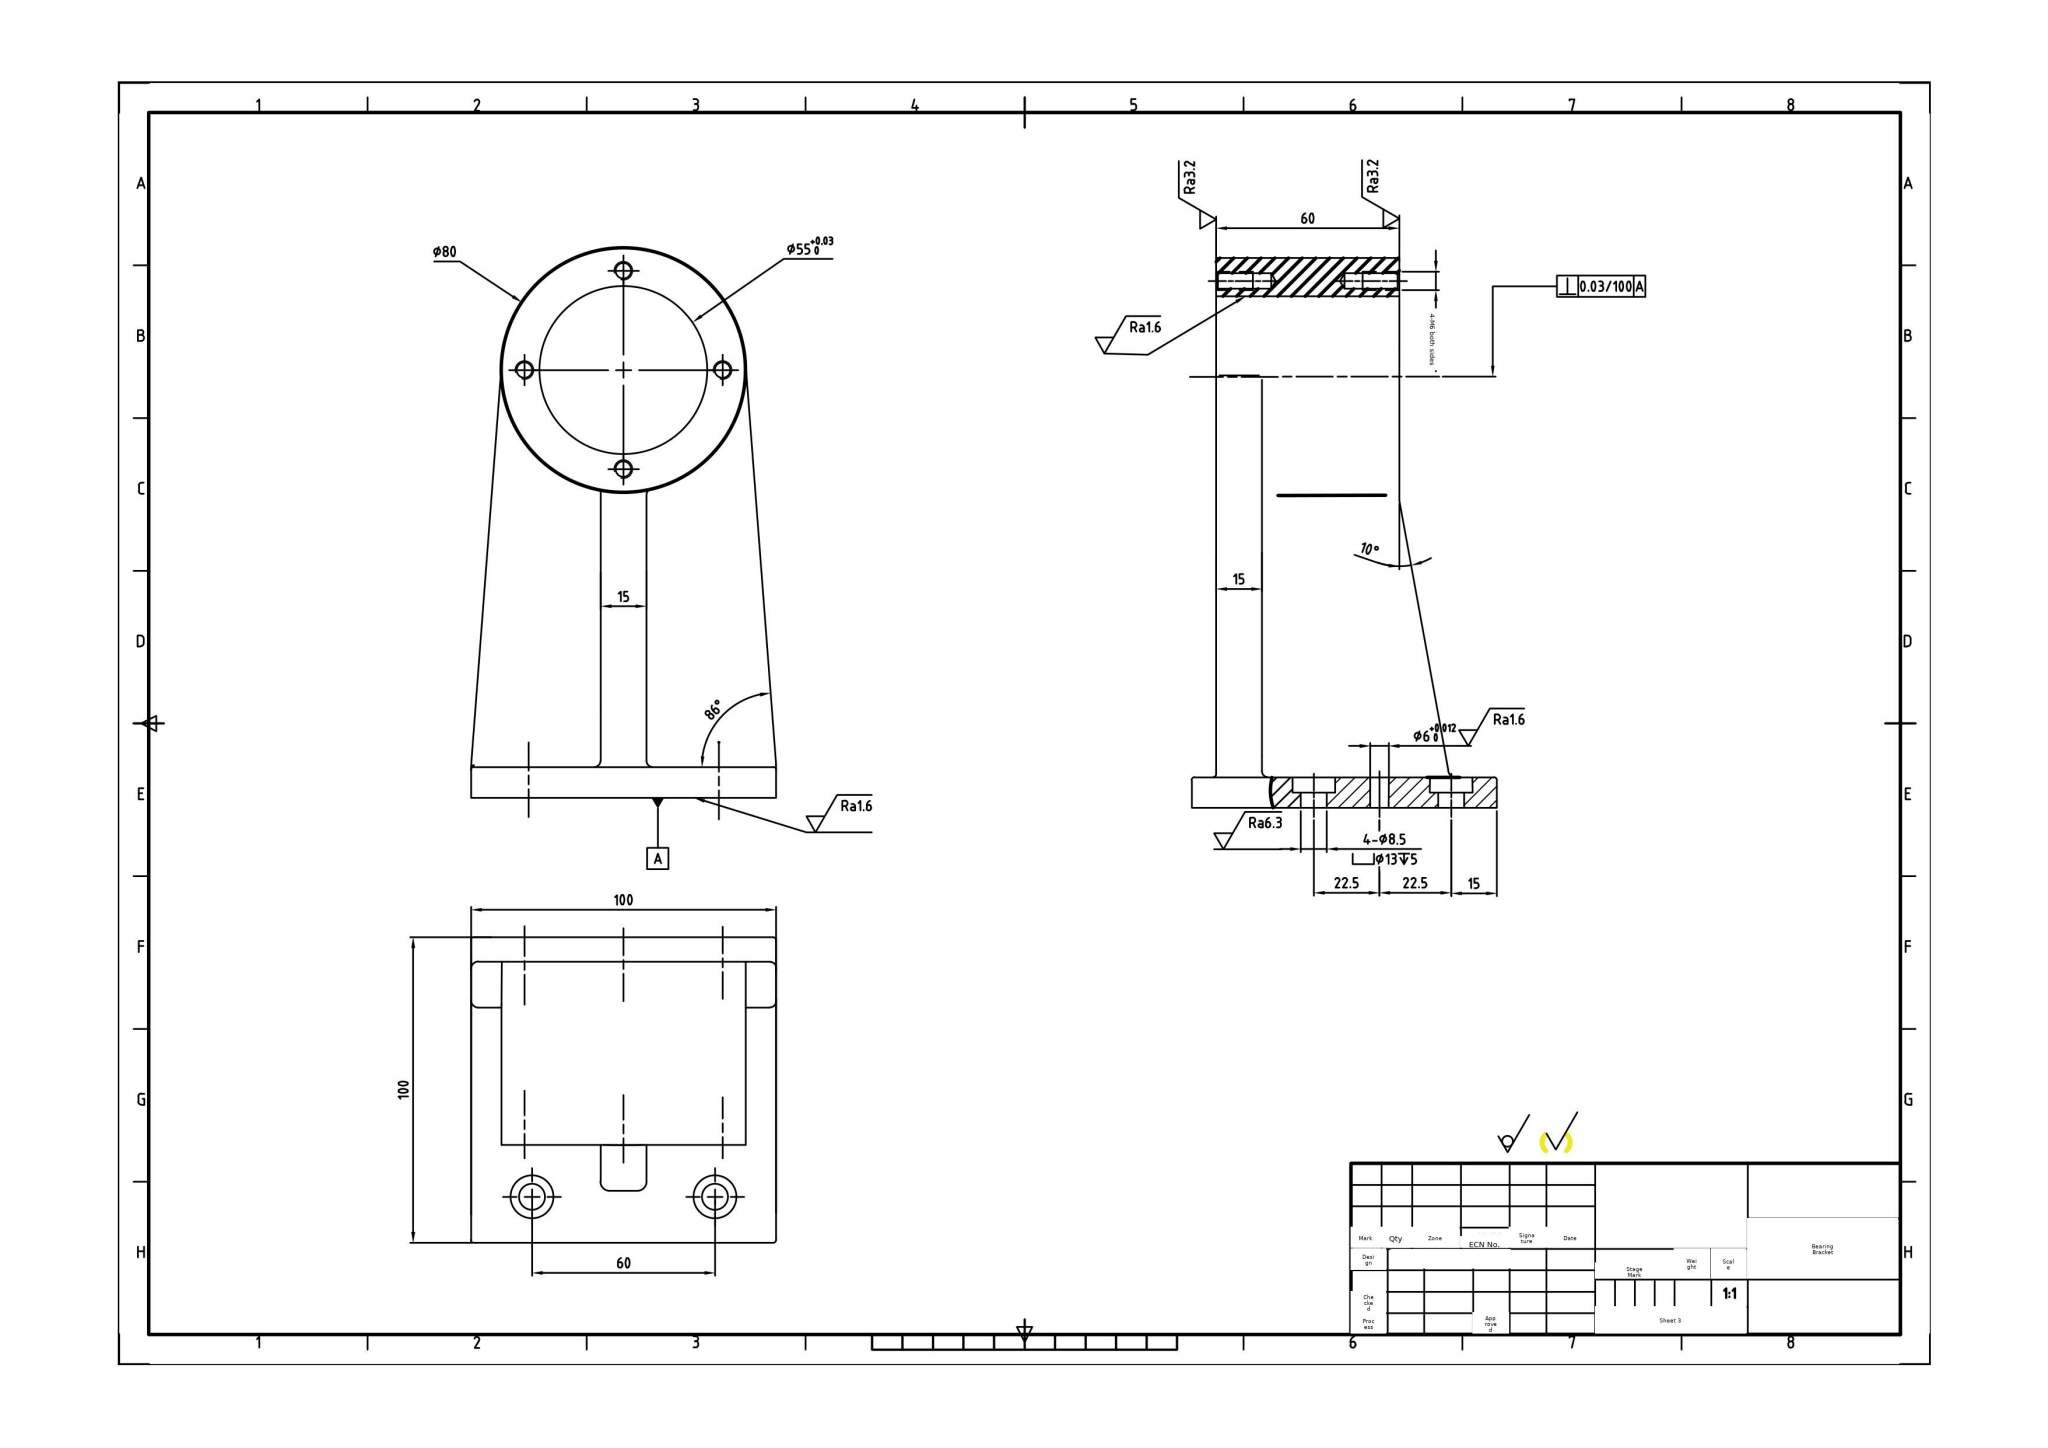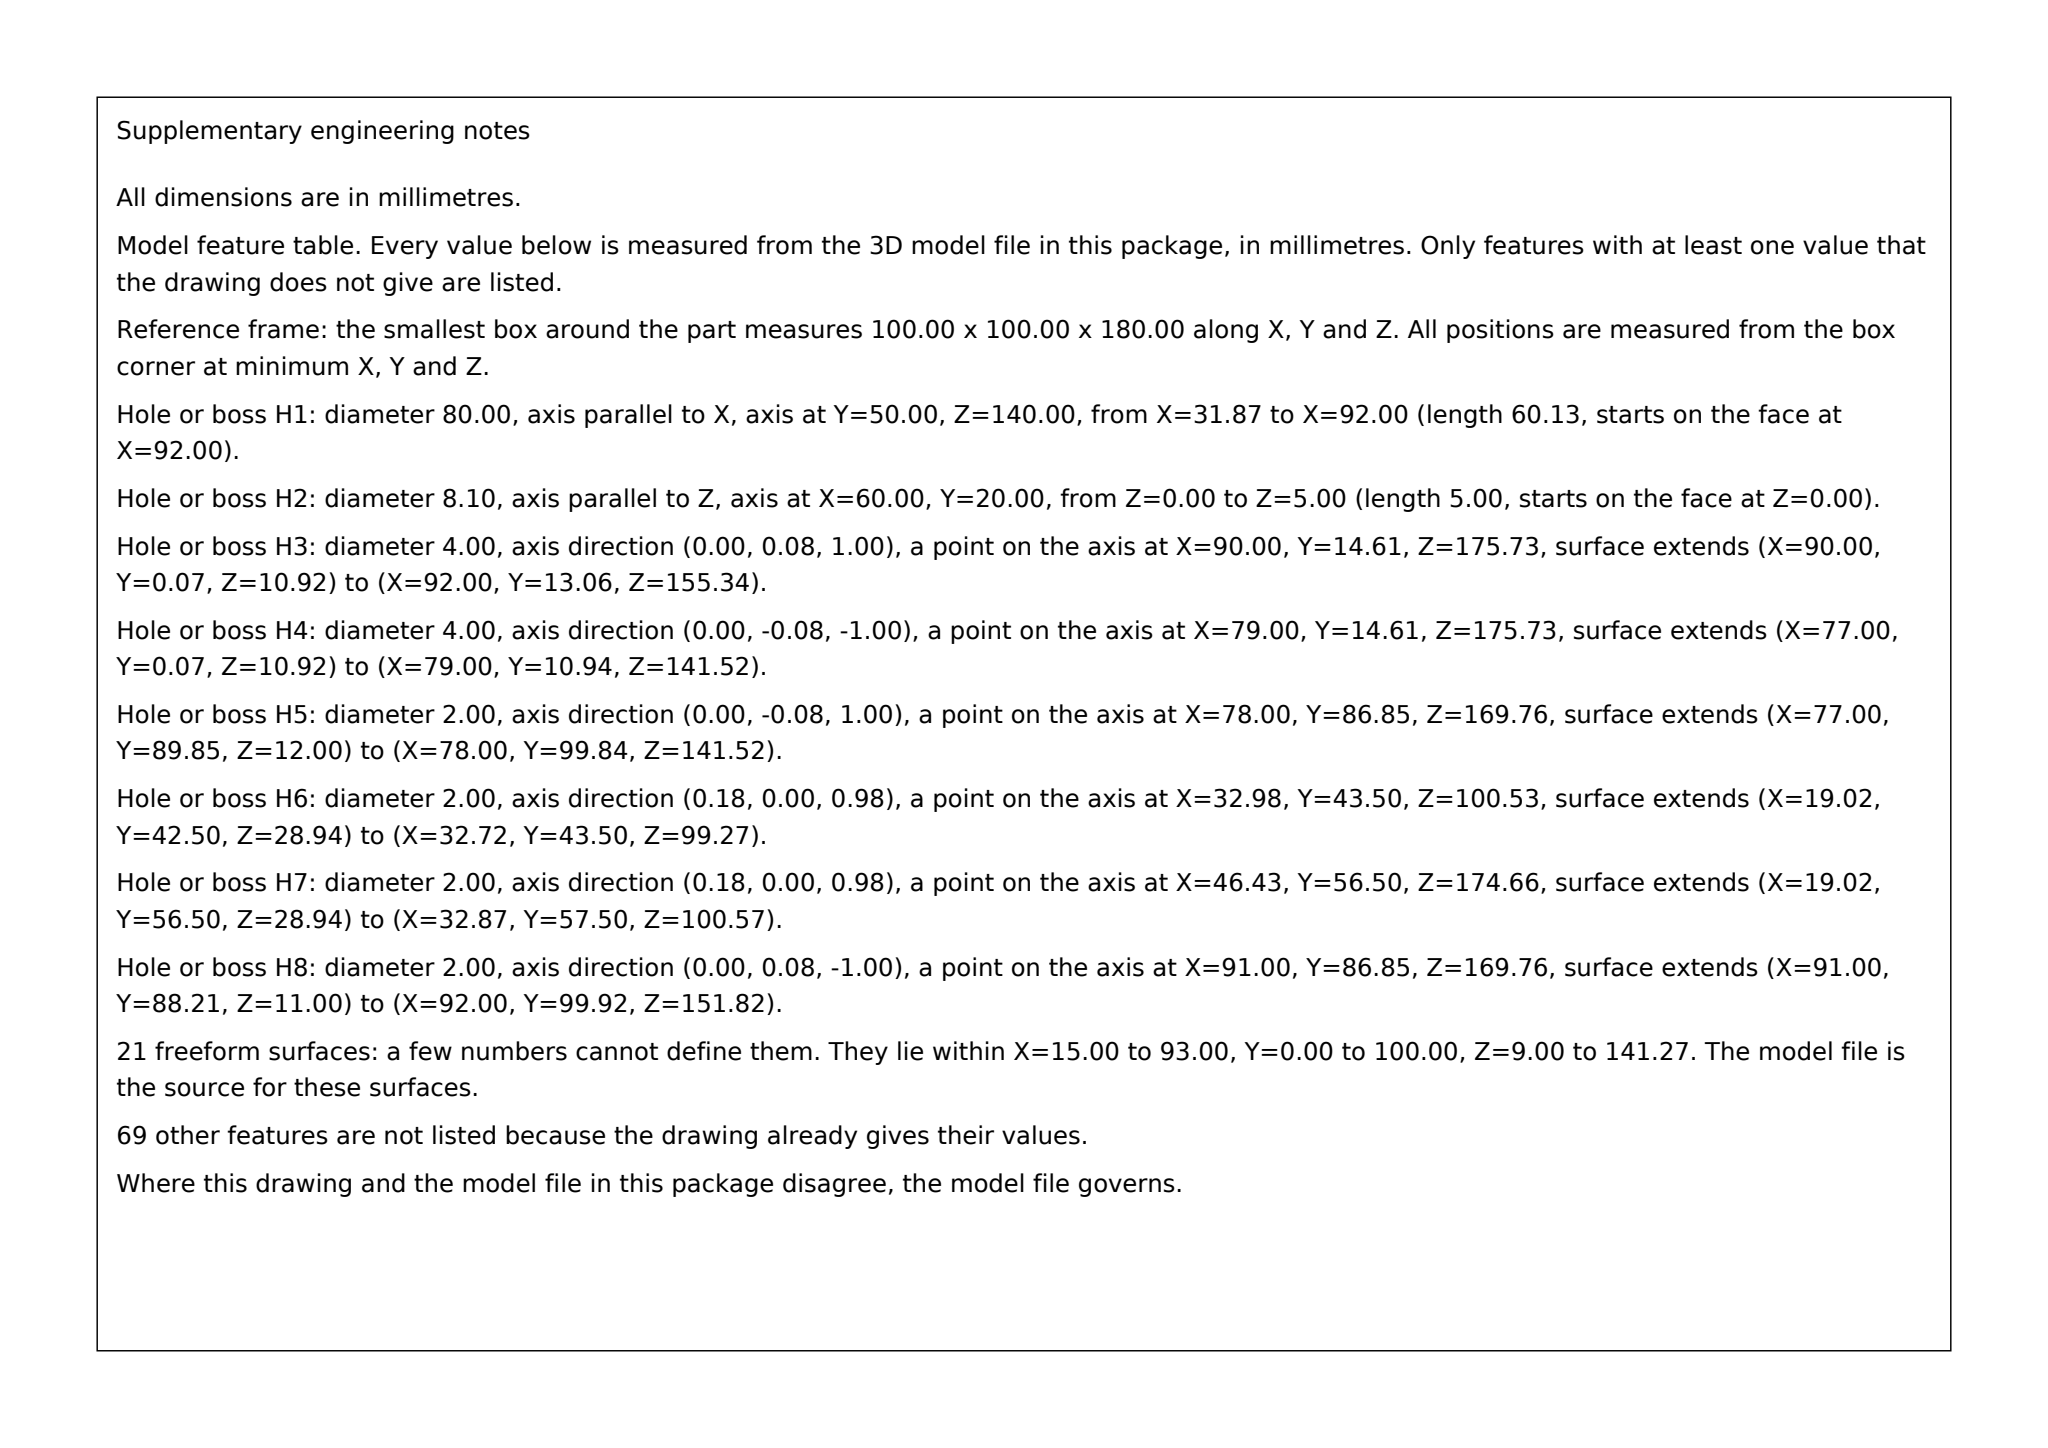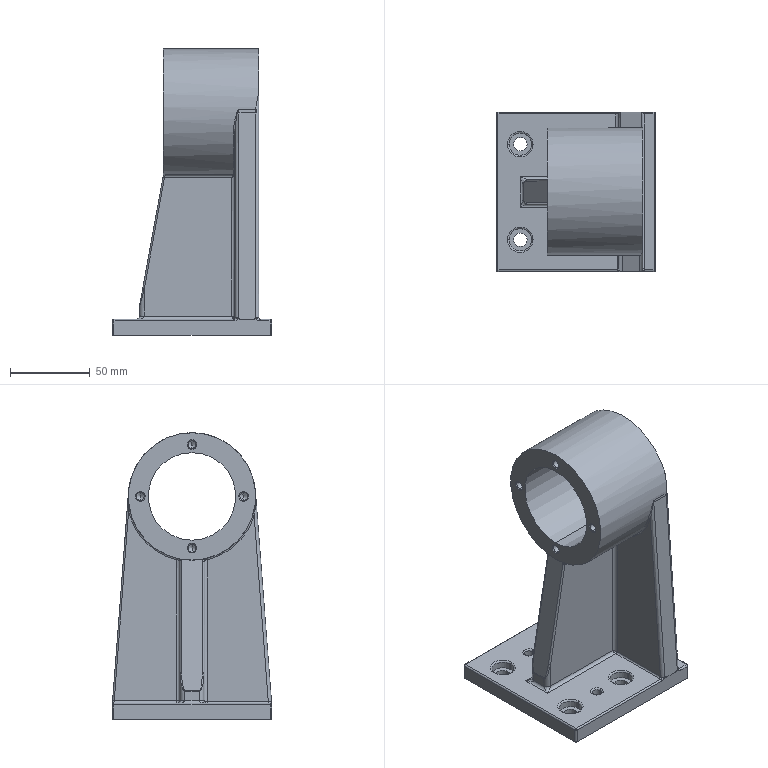Part | SolidWorks | mm | 1 solid | 168 faces | box 100 x 100 x 180 mm | volume 461259 mm3 | cylinder 71 | cone 32 | plane 23 | spline 21 | torus 16 | sphere 5 | commonest cylinder face diameters 2 x18 5 x16 4 x9 14 x8 6 x7 8.5 x6 80 x3 8.106 x2